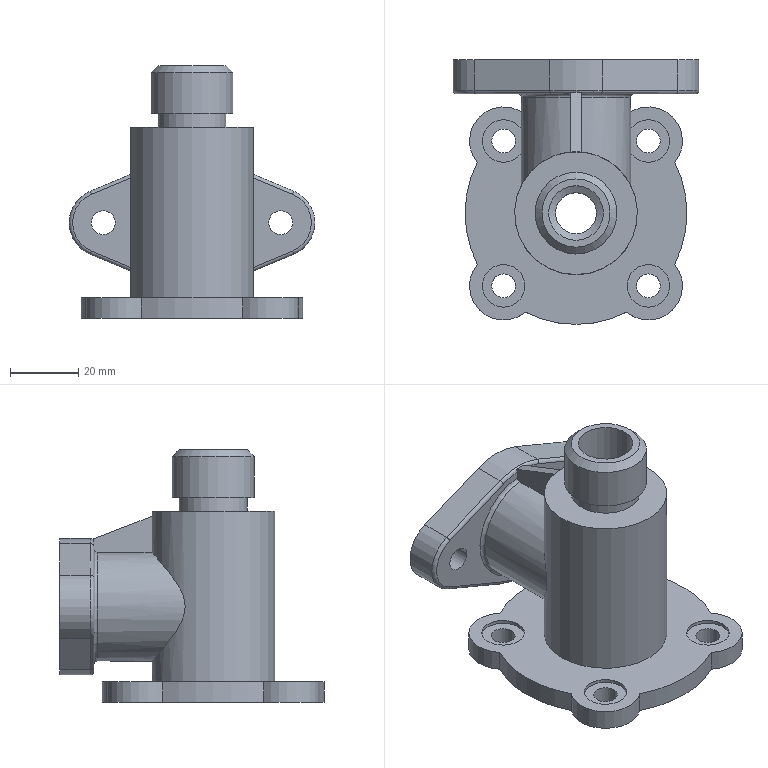Component | NX | UPPER_VALVE_BODY | 1 solid | 63 faces | volume 72991 mm3 | cylinder 35 | plane 20 | torus 5 | cone 3 | commonest cylinder face diameters 20 x7 7 x6 65 x4 2 x4 12.5 x4 40 x2 32 x1 12 x1